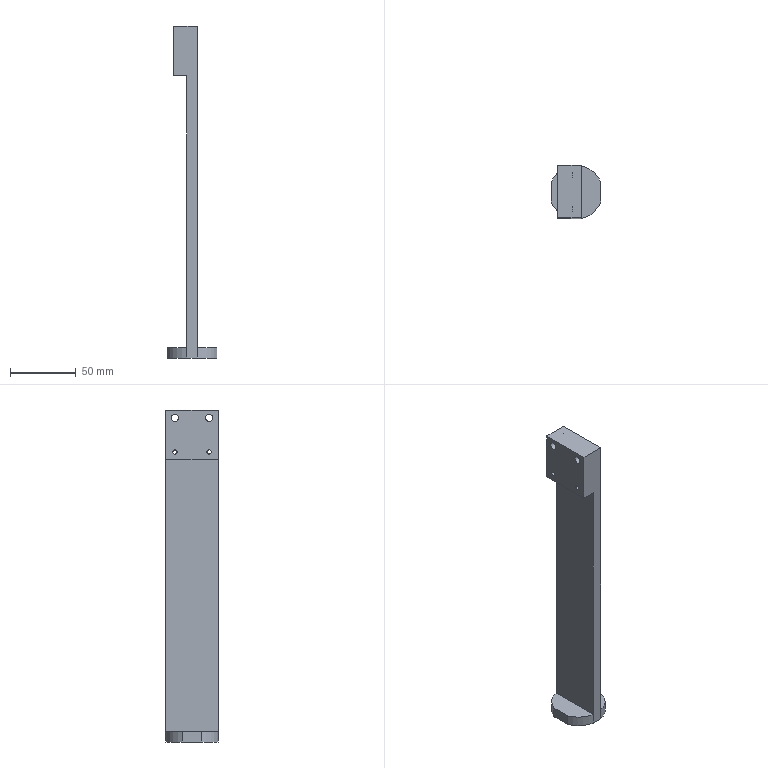Component | NX | PRESS_BODY | 1 solid | 28 faces | volume 100620 mm3 | plane 16 | cylinder 12 | commonest cylinder face diameters 40.792 x4 11 x4 5.5 x2 3.271 x2